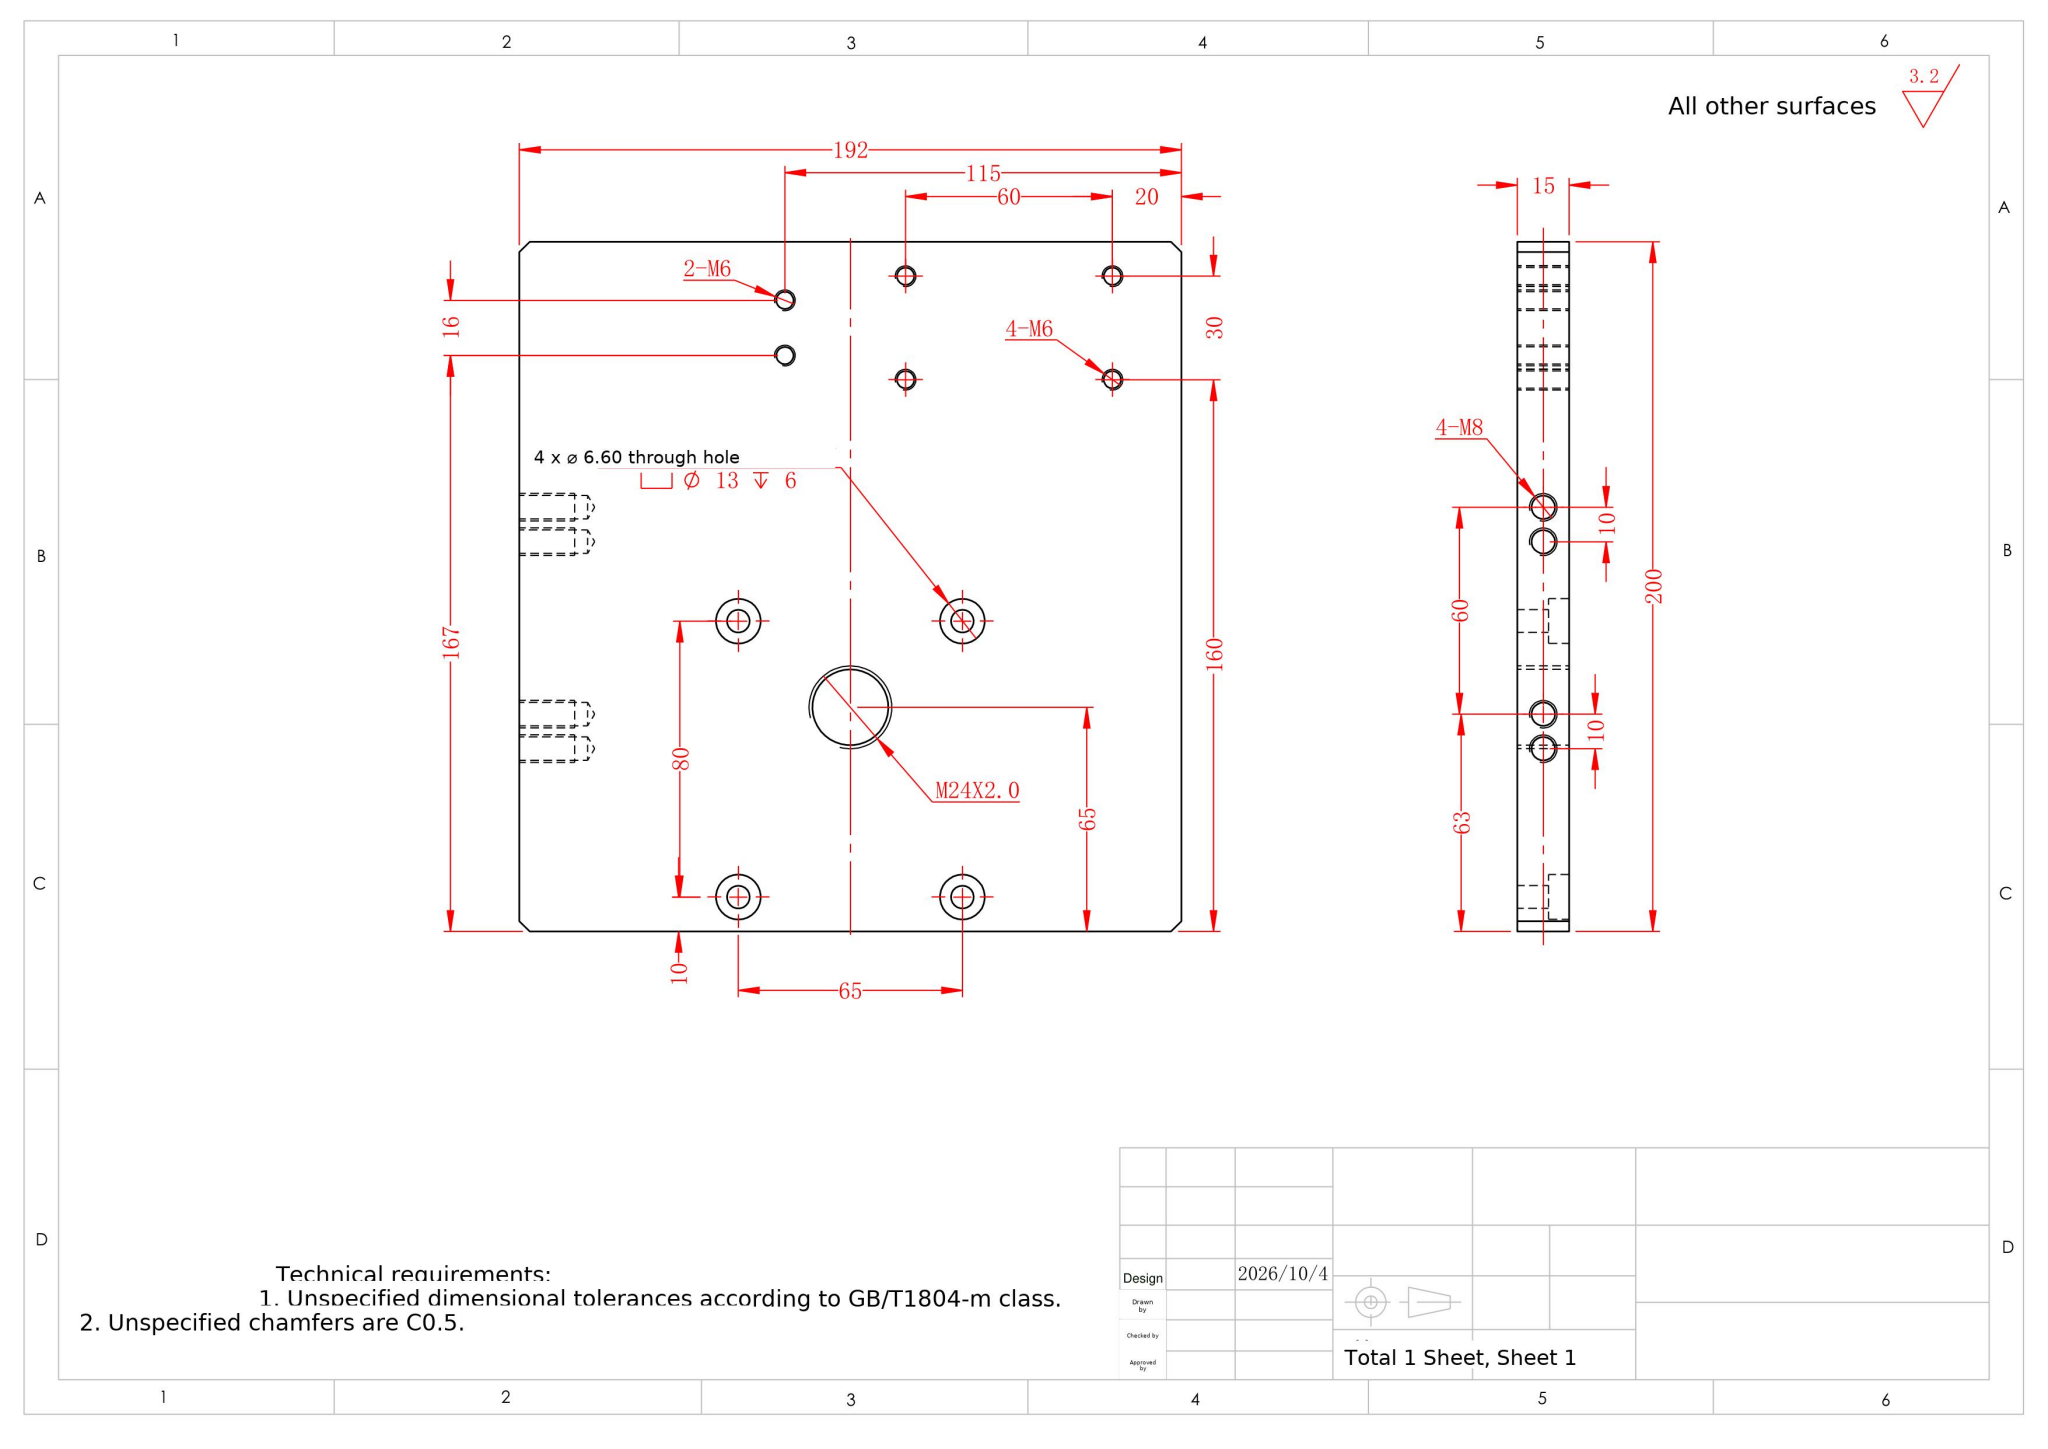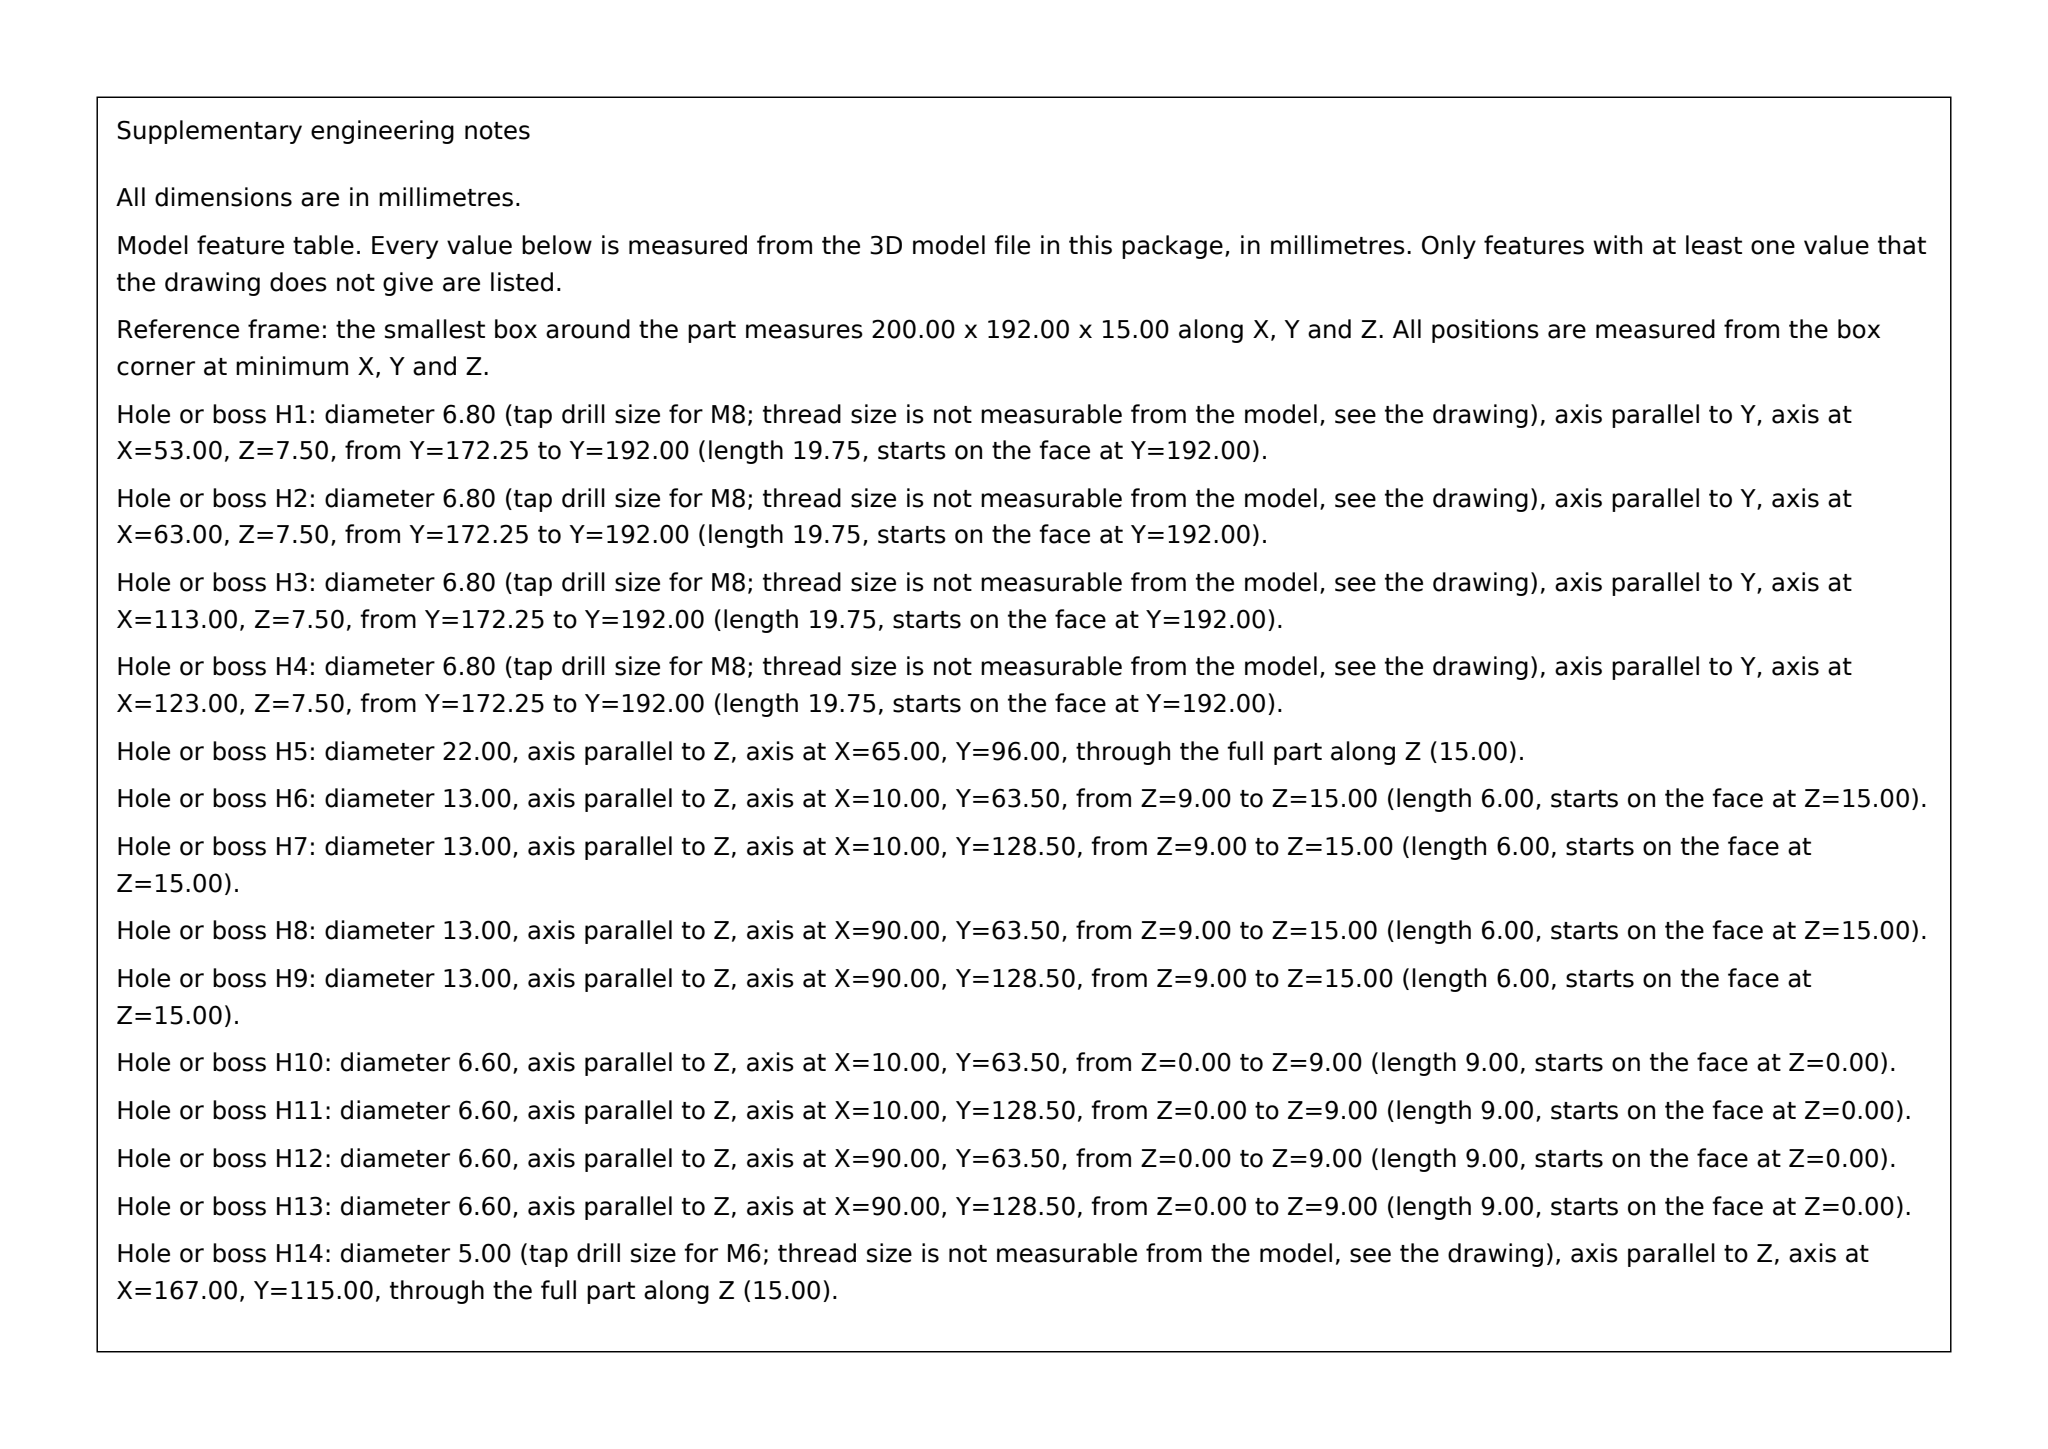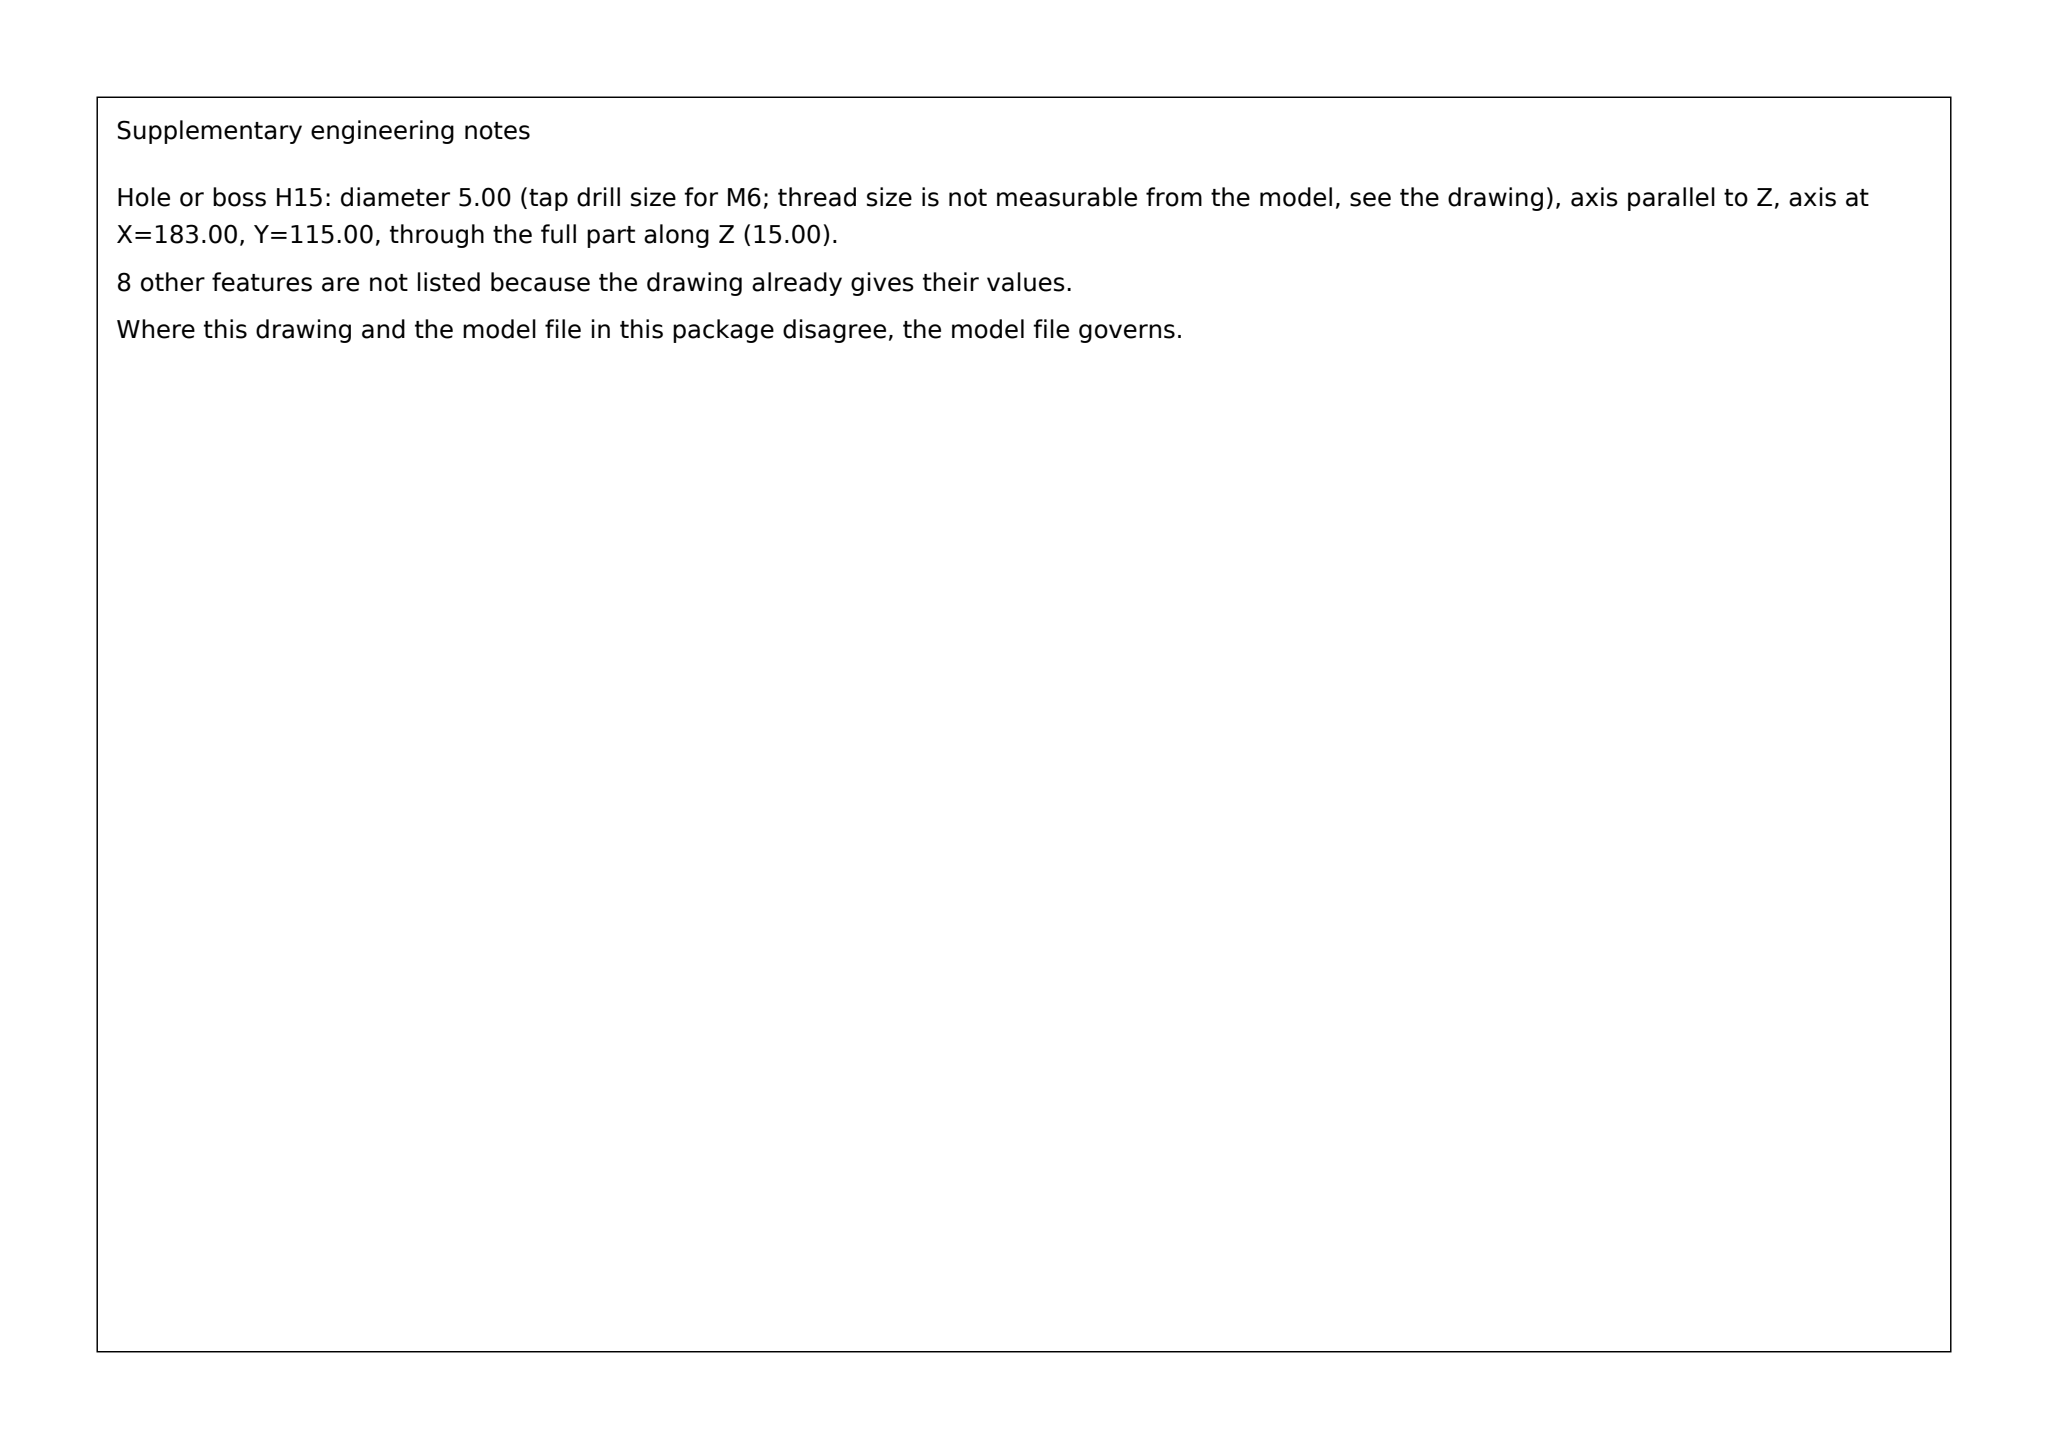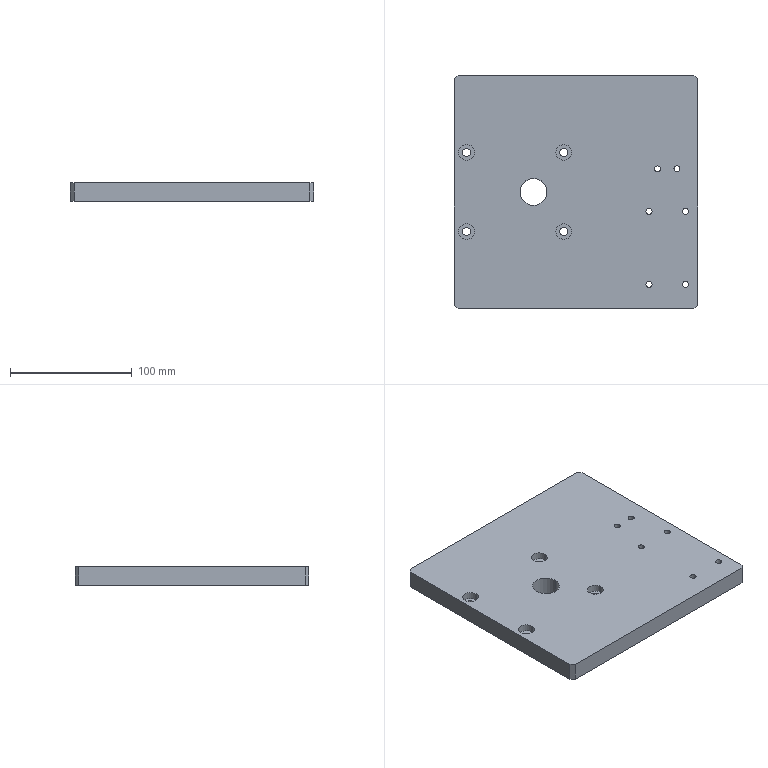Part | SolidWorks | mm | 1 solid | 60 faces | box 200 x 192 x 15 mm | volume 560876 mm3 | cylinder 38 | plane 14 | cone 8 | commonest cylinder face diameters 5 x12 6.8 x8 13 x8 6.6 x8 22 x2
build123d program:
from build123d import *

# Parameters (mm, degrees)
SKETCH1_W                                           = 200
SKETCH1_H                                           = 192
BOSS_EXTRUDE1_DEPTH                                 = 15
CYLINDRICAL_COUNTERSUNK_HOLE_FOR_M6_HEX_D           = 6.6
CYLINDRICAL_COUNTERSUNK_HOLE_FOR_M6_HEX_CBORE_D     = 13
CYLINDRICAL_COUNTERSUNK_HOLE_FOR_M6_HEX_CBORE_DEPTH = 6
M8_TAPPED_HOLE1_D                                   = 6.8
M8_TAPPED_HOLE1_DEPTH                               = 19.75
M8_TAPPED_HOLE1_TIP                                 = 2.043
M6_TAPPED_HOLE1_D                                   = 5
CHAMFER1_SIZE                                       = 3
M24X2_0_TAPPED_HOLE1_D                              = 22


with BuildPart() as part:
    # Sketch1 → Boss-Extrude1 (new body)
    with BuildSketch(Plane.XY):
        Rectangle(SKETCH1_W, SKETCH1_H)
    extrude(amount=BOSS_EXTRUDE1_DEPTH)

    # Cylindrical Countersunk Hole for M6 Hex (through all)
    with Locations(Plane.XY.offset(15)):
        with Locations((-90, 32.5), (-10, 32.5), (-10, -32.5), (-90, -32.5)):
            CounterBoreHole(CYLINDRICAL_COUNTERSUNK_HOLE_FOR_M6_HEX_D / 2, CYLINDRICAL_COUNTERSUNK_HOLE_FOR_M6_HEX_CBORE_D / 2, CYLINDRICAL_COUNTERSUNK_HOLE_FOR_M6_HEX_CBORE_DEPTH)

    # M8 Tapped Hole1
    with Locations(Plane(origin=(0, 96, 0), x_dir=(1, 0, 0), z_dir=(0, 1, 0))):
        with Locations((-37, -7.5), (23, -7.5), (13, -7.5), (-47, -7.5)):
            Hole(M8_TAPPED_HOLE1_D / 2, depth=M8_TAPPED_HOLE1_DEPTH)
            with Locations((0, 0, -(M8_TAPPED_HOLE1_DEPTH + M8_TAPPED_HOLE1_TIP / 2))):  # 118° drill point
                Cone(0, M8_TAPPED_HOLE1_D / 2, M8_TAPPED_HOLE1_TIP, mode=Mode.SUBTRACT)

    # M6 Tapped Hole1 (through all)
    with Locations(Plane.XY.offset(15)):
        with Locations((60, -76), (60, -16), (90, -16), (90, -76), (67, 19), (83, 19)):
            Hole(M6_TAPPED_HOLE1_D / 2)

    # Chamfer1
    chamfer1_edges = [part.edges().sort_by_distance(p)[0] for p in [
        (100, -96, 7.5),
        (-100, -96, 7.5),
        (-100, 96, 7.5),
        (100, 96, 7.5),
    ]]
    chamfer(chamfer1_edges, length=CHAMFER1_SIZE)

    # M24x2.0 Tapped Hole1 (through all)
    with Locations(Plane.XY.offset(15)):
        with Locations((-35, 0)):
            Hole(M24X2_0_TAPPED_HOLE1_D / 2)


solid = part.part